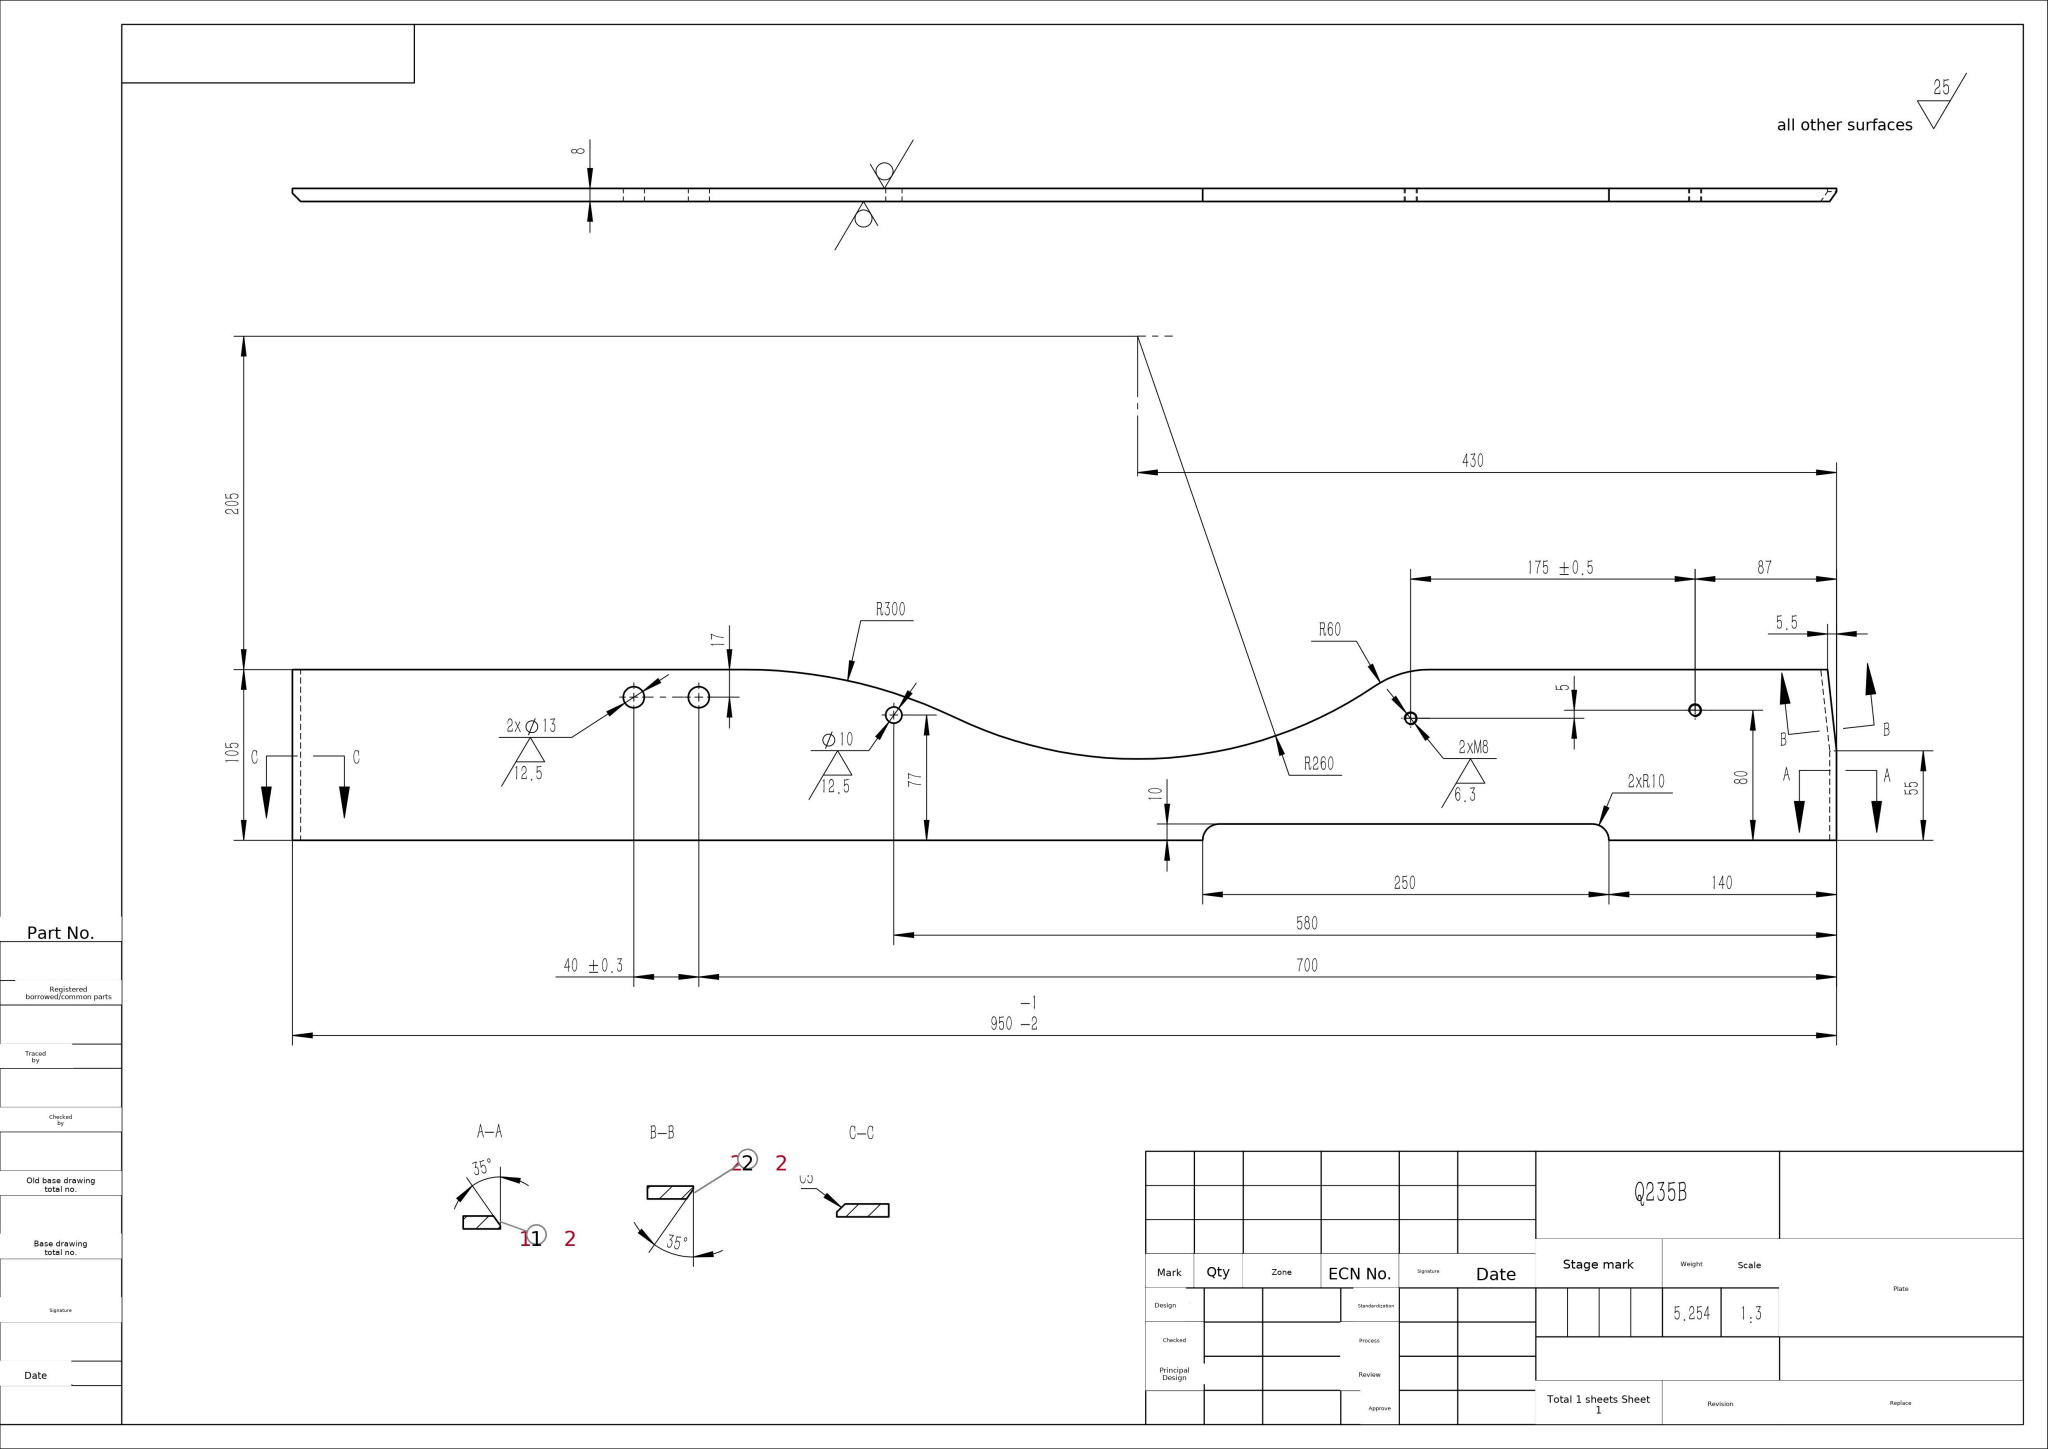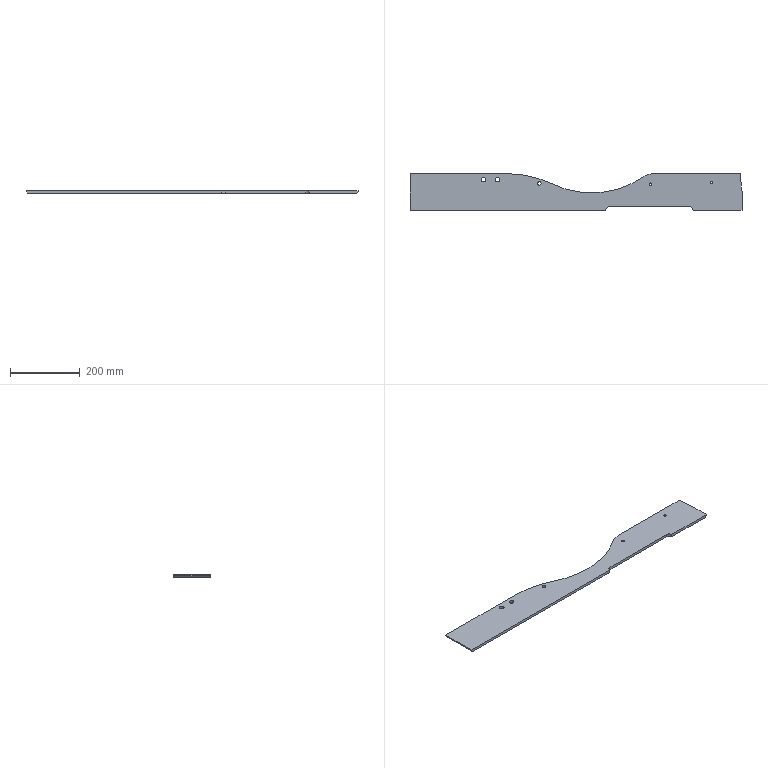Part | SolidWorks | mm | material Q235B | 1 solid | 28 faces | box 950 x 105 x 8 mm | volume 671051 mm3 | cylinder 15 | plane 13 | commonest cylinder face diameters 6.8 x4 13 x4 10 x2 20 x2 120 x1 520 x1 600 x1
build123d program:
from build123d import *
from OCP.BRepFilletAPI import BRepFilletAPI_MakeChamfer

# Parameters (mm, degrees)
SKETCH1_R           = 5
SKETCH1_R_2         = 6.5
BOSS_EXTRUDE1_DEPTH = 8
M8_TAPPED_HOLE1_D   = 6.8
CHAMFER1_SIZE       = 5
CHAMFER2_SIZE       = 6
CHAMFER2_SIZE2      = 4.201


with BuildPart() as part:
    # Sketch1 → Boss-Extrude1 (new body)
    with BuildSketch(Plane.XY):
        with BuildLine():
            Line((0, 0), (560, 0))
            ThreePointArc((560, 0), (562.929, 7.071), (570, 10))
            Line((570, 10), (800, 10))
            ThreePointArc((800, 10), (807.071, 7.071), (810, 0))
            Line((810, 0), (950, 0))
            Line((950, 0), (950, 55))
            Line((950, 55), (944.5, 105))
            Line((944.5, 105), (699.374, 105))
            ThreePointArc((699.374, 105), (681.785, 102.364), (665.741, 94.688))
            ThreePointArc((665.741, 94.688), (539.239, 50.713), (407.632, 75.536))
            ThreePointArc((407.632, 75.536), (344.458, 97.541), (277.977, 105))
            Line((277.977, 105), (0, 105))
            Line((0, 105), (0, 0))
        make_face()
        with Locations((370, 77)):
            Circle(SKETCH1_R, mode=Mode.SUBTRACT)
        with Locations((250, 88)):
            Circle(SKETCH1_R_2, mode=Mode.SUBTRACT)
        with Locations((210, 88)):
            Circle(SKETCH1_R_2, mode=Mode.SUBTRACT)
    extrude(amount=BOSS_EXTRUDE1_DEPTH)

    # M8 Tapped Hole1 (through all)
    with Locations(Plane(origin=(863, 80, 8), x_dir=(1, 0, 0), z_dir=(0, 0, 1))):
        with Locations((0, 0), (-175, -5)):
            Hole(M8_TAPPED_HOLE1_D / 2)

    # Chamfer1
    chamfer1_edges = [part.edges().sort_by_distance(p)[0] for p in [
        (0, 52.5, 0),
    ]]
    chamfer(chamfer1_edges, length=CHAMFER1_SIZE)

    # Chamfer2: one chamfer whose edges measure the first distance from different faces: ONE call of the kernel's chamfer builder (chamfer() names one face for all edges)
    chamfer2_edges_1 = [part.edges().sort_by_distance(p)[0] for p in [
        (947.25, 80, 0),
    ]]
    chamfer2_side_1 = [part.faces().sort_by_distance(p)[0] for p in [
        (947.25, 80, 4),
    ]]
    chamfer2_edges_2 = [part.edges().sort_by_distance(p)[0] for p in [
        (950, 27.5, 0),
    ]]
    chamfer2_side_2 = [part.faces().sort_by_distance(p)[0] for p in [
        (950, 27.5, 4),
    ]]
    chamfer2 = BRepFilletAPI_MakeChamfer(part.part.solid().wrapped)
    for e in chamfer2_edges_1:
        chamfer2.Add(CHAMFER2_SIZE, CHAMFER2_SIZE2, e.wrapped, chamfer2_side_1[0].wrapped)  # the first distance lies on this face
    for e in chamfer2_edges_2:
        chamfer2.Add(CHAMFER2_SIZE, CHAMFER2_SIZE2, e.wrapped, chamfer2_side_2[0].wrapped)  # the first distance lies on this face
    add(Compound.cast(chamfer2.Shape()), mode=Mode.REPLACE)


solid = part.part
STEP:
#1=CARTESIAN_POINT('',(866.4,80.,0.));
#2=VERTEX_POINT('',#1);
#3=CARTESIAN_POINT('',(859.6,80.,0.));
#4=VERTEX_POINT('',#3);
#5=CARTESIAN_POINT('',(863.,80.,0.));
#6=DIRECTION('',(0.,0.,-1.));
#7=DIRECTION('',(-1.,0.,0.));
#8=AXIS2_PLACEMENT_3D('',#5,#6,#7);
#9=CIRCLE('',#8,3.4);
#10=EDGE_CURVE('',#2,#4,#9,.T.);
#11=ORIENTED_EDGE('',*,*,#10,.T.);
#12=CARTESIAN_POINT('',(859.6,80.,8.));
#13=VERTEX_POINT('',#12);
#14=CARTESIAN_POINT('',(859.6,80.,8.));
#15=DIRECTION('',(0.,0.,1.));
#16=VECTOR('',#15,1000.);
#17=LINE('',#14,#16);
#18=EDGE_CURVE('',#4,#13,#17,.T.);
#19=ORIENTED_EDGE('',*,*,#18,.T.);
#20=CARTESIAN_POINT('',(866.4,80.,8.));
#21=VERTEX_POINT('',#20);
#22=CARTESIAN_POINT('',(863.,80.,8.));
#23=DIRECTION('',(0.,0.,1.));
#24=DIRECTION('',(1.,0.,0.));
#25=AXIS2_PLACEMENT_3D('',#22,#23,#24);
#26=CIRCLE('',#25,3.4);
#27=EDGE_CURVE('',#13,#21,#26,.T.);
#28=ORIENTED_EDGE('',*,*,#27,.T.);
#29=CARTESIAN_POINT('',(866.4,80.,8.));
#30=DIRECTION('',(0.,0.,1.));
#31=VECTOR('',#30,1000.);
#32=LINE('',#29,#31);
#33=EDGE_CURVE('',#2,#21,#32,.T.);
#34=ORIENTED_EDGE('',*,*,#33,.F.);
#35=EDGE_LOOP('',(#11,#19,#28,#34));
#36=FACE_OUTER_BOUND('',#35,.T.);
#37=CARTESIAN_POINT('',(863.,80.,8.));
#38=DIRECTION('',(0.,0.,1.));
#39=DIRECTION('',(1.,0.,0.));
#40=AXIS2_PLACEMENT_3D('',#37,#38,#39);
#41=CYLINDRICAL_SURFACE('',#40,3.4);
#42=ADVANCED_FACE('',(#36),#41,.F.);
#43=CARTESIAN_POINT('',(691.4,75.,0.));
#44=VERTEX_POINT('',#43);
#45=CARTESIAN_POINT('',(684.6,75.,0.));
#46=VERTEX_POINT('',#45);
#47=CARTESIAN_POINT('',(688.,75.,0.));
#48=DIRECTION('',(0.,0.,-1.));
#49=DIRECTION('',(-1.,0.,0.));
#50=AXIS2_PLACEMENT_3D('',#47,#48,#49);
#51=CIRCLE('',#50,3.4);
#52=EDGE_CURVE('',#44,#46,#51,.T.);
#53=ORIENTED_EDGE('',*,*,#52,.T.);
#54=CARTESIAN_POINT('',(684.6,75.,8.));
#55=VERTEX_POINT('',#54);
#56=CARTESIAN_POINT('',(684.6,75.,8.));
#57=DIRECTION('',(0.,0.,1.));
#58=VECTOR('',#57,1000.);
#59=LINE('',#56,#58);
#60=EDGE_CURVE('',#46,#55,#59,.T.);
#61=ORIENTED_EDGE('',*,*,#60,.T.);
#62=CARTESIAN_POINT('',(691.4,75.,8.));
#63=VERTEX_POINT('',#62);
#64=CARTESIAN_POINT('',(688.,75.,8.));
#65=DIRECTION('',(0.,0.,1.));
#66=DIRECTION('',(1.,0.,0.));
#67=AXIS2_PLACEMENT_3D('',#64,#65,#66);
#68=CIRCLE('',#67,3.4);
#69=EDGE_CURVE('',#55,#63,#68,.T.);
#70=ORIENTED_EDGE('',*,*,#69,.T.);
#71=CARTESIAN_POINT('',(691.4,75.,8.));
#72=DIRECTION('',(0.,0.,1.));
#73=VECTOR('',#72,1000.);
#74=LINE('',#71,#73);
#75=EDGE_CURVE('',#44,#63,#74,.T.);
#76=ORIENTED_EDGE('',*,*,#75,.F.);
#77=EDGE_LOOP('',(#53,#61,#70,#76));
#78=FACE_OUTER_BOUND('',#77,.T.);
#79=CARTESIAN_POINT('',(688.,75.,8.));
#80=DIRECTION('',(0.,0.,1.));
#81=DIRECTION('',(1.,0.,0.));
#82=AXIS2_PLACEMENT_3D('',#79,#80,#81);
#83=CYLINDRICAL_SURFACE('',#82,3.4);
#84=ADVANCED_FACE('',(#78),#83,.F.);
#85=CARTESIAN_POINT('',(203.5,88.,8.));
#86=VERTEX_POINT('',#85);
#87=CARTESIAN_POINT('',(216.5,88.,8.));
#88=VERTEX_POINT('',#87);
#89=CARTESIAN_POINT('',(210.,88.,8.));
#90=DIRECTION('',(0.,0.,1.));
#91=DIRECTION('',(1.,0.,0.));
#92=AXIS2_PLACEMENT_3D('',#89,#90,#91);
#93=CIRCLE('',#92,6.5);
#94=EDGE_CURVE('',#86,#88,#93,.T.);
#95=ORIENTED_EDGE('',*,*,#94,.T.);
#96=CARTESIAN_POINT('',(216.5,88.,0.));
#97=VERTEX_POINT('',#96);
#98=CARTESIAN_POINT('',(216.5,88.,8.));
#99=DIRECTION('',(0.,0.,-1.));
#100=VECTOR('',#99,1000.);
#101=LINE('',#98,#100);
#102=EDGE_CURVE('',#88,#97,#101,.T.);
#103=ORIENTED_EDGE('',*,*,#102,.T.);
#104=CARTESIAN_POINT('',(203.5,88.,0.));
#105=VERTEX_POINT('',#104);
#106=CARTESIAN_POINT('',(210.,88.,0.));
#107=DIRECTION('',(0.,0.,1.));
#108=DIRECTION('',(1.,0.,0.));
#109=AXIS2_PLACEMENT_3D('',#106,#107,#108);
#110=CIRCLE('',#109,6.5);
#111=EDGE_CURVE('',#105,#97,#110,.T.);
#112=ORIENTED_EDGE('',*,*,#111,.F.);
#113=CARTESIAN_POINT('',(203.5,88.,8.));
#114=DIRECTION('',(0.,0.,-1.));
#115=VECTOR('',#114,1000.);
#116=LINE('',#113,#115);
#117=EDGE_CURVE('',#86,#105,#116,.T.);
#118=ORIENTED_EDGE('',*,*,#117,.F.);
#119=EDGE_LOOP('',(#95,#103,#112,#118));
#120=FACE_OUTER_BOUND('',#119,.T.);
#121=CARTESIAN_POINT('',(210.,88.,8.));
#122=DIRECTION('',(0.,0.,-1.));
#123=DIRECTION('',(-1.,0.,0.));
#124=AXIS2_PLACEMENT_3D('',#121,#122,#123);
#125=CYLINDRICAL_SURFACE('',#124,6.5);
#126=ADVANCED_FACE('',(#120),#125,.F.);
#127=CARTESIAN_POINT('',(243.5,88.,8.));
#128=VERTEX_POINT('',#127);
#129=CARTESIAN_POINT('',(256.5,88.,8.));
#130=VERTEX_POINT('',#129);
#131=CARTESIAN_POINT('',(250.,88.,8.));
#132=DIRECTION('',(0.,0.,1.));
#133=DIRECTION('',(1.,0.,0.));
#134=AXIS2_PLACEMENT_3D('',#131,#132,#133);
#135=CIRCLE('',#134,6.5);
#136=EDGE_CURVE('',#128,#130,#135,.T.);
#137=ORIENTED_EDGE('',*,*,#136,.T.);
#138=CARTESIAN_POINT('',(256.5,88.,0.));
#139=VERTEX_POINT('',#138);
#140=CARTESIAN_POINT('',(256.5,88.,8.));
#141=DIRECTION('',(0.,0.,-1.));
#142=VECTOR('',#141,1000.);
#143=LINE('',#140,#142);
#144=EDGE_CURVE('',#130,#139,#143,.T.);
#145=ORIENTED_EDGE('',*,*,#144,.T.);
#146=CARTESIAN_POINT('',(243.5,88.,0.));
#147=VERTEX_POINT('',#146);
#148=CARTESIAN_POINT('',(250.,88.,0.));
#149=DIRECTION('',(0.,0.,1.));
#150=DIRECTION('',(1.,0.,0.));
#151=AXIS2_PLACEMENT_3D('',#148,#149,#150);
#152=CIRCLE('',#151,6.5);
#153=EDGE_CURVE('',#147,#139,#152,.T.);
#154=ORIENTED_EDGE('',*,*,#153,.F.);
#155=CARTESIAN_POINT('',(243.5,88.,8.));
#156=DIRECTION('',(0.,0.,-1.));
#157=VECTOR('',#156,1000.);
#158=LINE('',#155,#157);
#159=EDGE_CURVE('',#128,#147,#158,.T.);
#160=ORIENTED_EDGE('',*,*,#159,.F.);
#161=EDGE_LOOP('',(#137,#145,#154,#160));
#162=FACE_OUTER_BOUND('',#161,.T.);
#163=CARTESIAN_POINT('',(250.,88.,8.));
#164=DIRECTION('',(0.,0.,-1.));
#165=DIRECTION('',(-1.,0.,0.));
#166=AXIS2_PLACEMENT_3D('',#163,#164,#165);
#167=CYLINDRICAL_SURFACE('',#166,6.5);
#168=ADVANCED_FACE('',(#162),#167,.F.);
#169=CARTESIAN_POINT('',(365.,77.,8.));
#170=VERTEX_POINT('',#169);
#171=CARTESIAN_POINT('',(375.,77.,8.));
#172=VERTEX_POINT('',#171);
#173=CARTESIAN_POINT('',(370.,77.,8.));
#174=DIRECTION('',(0.,0.,1.));
#175=DIRECTION('',(1.,0.,0.));
#176=AXIS2_PLACEMENT_3D('',#173,#174,#175);
#177=CIRCLE('',#176,5.);
#178=EDGE_CURVE('',#170,#172,#177,.T.);
#179=ORIENTED_EDGE('',*,*,#178,.T.);
#180=CARTESIAN_POINT('',(375.,77.,0.));
#181=VERTEX_POINT('',#180);
#182=CARTESIAN_POINT('',(375.,77.,8.));
#183=DIRECTION('',(0.,0.,-1.));
#184=VECTOR('',#183,1000.);
#185=LINE('',#182,#184);
#186=EDGE_CURVE('',#172,#181,#185,.T.);
#187=ORIENTED_EDGE('',*,*,#186,.T.);
#188=CARTESIAN_POINT('',(365.,77.,0.));
#189=VERTEX_POINT('',#188);
#190=CARTESIAN_POINT('',(370.,77.,0.));
#191=DIRECTION('',(0.,0.,1.));
#192=DIRECTION('',(1.,0.,0.));
#193=AXIS2_PLACEMENT_3D('',#190,#191,#192);
#194=CIRCLE('',#193,5.);
#195=EDGE_CURVE('',#189,#181,#194,.T.);
#196=ORIENTED_EDGE('',*,*,#195,.F.);
#197=CARTESIAN_POINT('',(365.,77.,8.));
#198=DIRECTION('',(0.,0.,-1.));
#199=VECTOR('',#198,1000.);
#200=LINE('',#197,#199);
#201=EDGE_CURVE('',#170,#189,#200,.T.);
#202=ORIENTED_EDGE('',*,*,#201,.F.);
#203=EDGE_LOOP('',(#179,#187,#196,#202));
#204=FACE_OUTER_BOUND('',#203,.T.);
#205=CARTESIAN_POINT('',(370.,77.,8.));
#206=DIRECTION('',(0.,0.,-1.));
#207=DIRECTION('',(-1.,0.,0.));
#208=AXIS2_PLACEMENT_3D('',#205,#206,#207);
#209=CYLINDRICAL_SURFACE('',#208,5.);
#210=ADVANCED_FACE('',(#204),#209,.F.);
#211=CARTESIAN_POINT('',(0.,105.,8.));
#212=VERTEX_POINT('',#211);
#213=CARTESIAN_POINT('',(0.,0.,8.));
#214=VERTEX_POINT('',#213);
#215=CARTESIAN_POINT('',(0.,105.,8.));
#216=DIRECTION('',(0.,-1.,0.));
#217=VECTOR('',#216,1000.);
#218=LINE('',#215,#217);
#219=EDGE_CURVE('',#212,#214,#218,.T.);
#220=ORIENTED_EDGE('',*,*,#219,.T.);
#221=CARTESIAN_POINT('',(560.,0.,8.));
#222=VERTEX_POINT('',#221);
#223=CARTESIAN_POINT('',(0.,0.,8.));
#224=DIRECTION('',(1.,0.,0.));
#225=VECTOR('',#224,1000.);
#226=LINE('',#223,#225);
#227=EDGE_CURVE('',#214,#222,#226,.T.);
#228=ORIENTED_EDGE('',*,*,#227,.T.);
#229=CARTESIAN_POINT('',(570.,10.,8.));
#230=VERTEX_POINT('',#229);
#231=CARTESIAN_POINT('',(570.,0.,8.));
#232=DIRECTION('',(0.,0.,-1.));
#233=DIRECTION('',(-1.,0.,0.));
#234=AXIS2_PLACEMENT_3D('',#231,#232,#233);
#235=CIRCLE('',#234,10.);
#236=EDGE_CURVE('',#222,#230,#235,.T.);
#237=ORIENTED_EDGE('',*,*,#236,.T.);
#238=CARTESIAN_POINT('',(800.,10.,8.));
#239=VERTEX_POINT('',#238);
#240=CARTESIAN_POINT('',(570.,10.,8.));
#241=DIRECTION('',(1.,0.,0.));
#242=VECTOR('',#241,1000.);
#243=LINE('',#240,#242);
#244=EDGE_CURVE('',#230,#239,#243,.T.);
#245=ORIENTED_EDGE('',*,*,#244,.T.);
#246=CARTESIAN_POINT('',(810.,0.,8.));
#247=VERTEX_POINT('',#246);
#248=CARTESIAN_POINT('',(800.,-0.,8.));
#249=DIRECTION('',(0.,0.,-1.));
#250=DIRECTION('',(1.,0.,0.));
#251=AXIS2_PLACEMENT_3D('',#248,#249,#250);
#252=CIRCLE('',#251,10.);
#253=EDGE_CURVE('',#239,#247,#252,.T.);
#254=ORIENTED_EDGE('',*,*,#253,.T.);
#255=CARTESIAN_POINT('',(950.,0.,8.));
#256=VERTEX_POINT('',#255);
#257=CARTESIAN_POINT('',(810.,0.,8.));
#258=DIRECTION('',(1.,0.,0.));
#259=VECTOR('',#258,1000.);
#260=LINE('',#257,#259);
#261=EDGE_CURVE('',#247,#256,#260,.T.);
#262=ORIENTED_EDGE('',*,*,#261,.T.);
#263=CARTESIAN_POINT('',(950.,55.,8.));
#264=VERTEX_POINT('',#263);
#265=CARTESIAN_POINT('',(950.,0.,8.));
#266=DIRECTION('',(0.,1.,0.));
#267=VECTOR('',#266,1000.);
#268=LINE('',#265,#267);
#269=EDGE_CURVE('',#256,#264,#268,.T.);
#270=ORIENTED_EDGE('',*,*,#269,.T.);
#271=CARTESIAN_POINT('',(944.5,105.,8.));
#272=VERTEX_POINT('',#271);
#273=CARTESIAN_POINT('',(950.,55.,8.));
#274=DIRECTION('',(-0.1093,0.994,0.));
#275=VECTOR('',#274,1000.);
#276=LINE('',#273,#275);
#277=EDGE_CURVE('',#264,#272,#276,.T.);
#278=ORIENTED_EDGE('',*,*,#277,.T.);
#279=CARTESIAN_POINT('',(699.374,105.,8.));
#280=VERTEX_POINT('',#279);
#281=CARTESIAN_POINT('',(944.5,105.,8.));
#282=DIRECTION('',(-1.,-0.,0.));
#283=VECTOR('',#282,1000.);
#284=LINE('',#281,#283);
#285=EDGE_CURVE('',#272,#280,#284,.T.);
#286=ORIENTED_EDGE('',*,*,#285,.T.);
#287=CARTESIAN_POINT('',(665.741,94.687,8.));
#288=VERTEX_POINT('',#287);
#289=CARTESIAN_POINT('',(699.374,45.,8.));
#290=DIRECTION('',(0.,0.,1.));
#291=DIRECTION('',(-1.,0.,0.));
#292=AXIS2_PLACEMENT_3D('',#289,#290,#291);
#293=CIRCLE('',#292,60.);
#294=EDGE_CURVE('',#280,#288,#293,.T.);
#295=ORIENTED_EDGE('',*,*,#294,.T.);
#296=CARTESIAN_POINT('',(407.632,75.536,8.));
#297=VERTEX_POINT('',#296);
#298=CARTESIAN_POINT('',(520.,310.,8.));
#299=DIRECTION('',(0.,0.,-1.));
#300=DIRECTION('',(1.,0.,0.));
#301=AXIS2_PLACEMENT_3D('',#298,#299,#300);
#302=CIRCLE('',#301,260.);
#303=EDGE_CURVE('',#288,#297,#302,.T.);
#304=ORIENTED_EDGE('',*,*,#303,.T.);
#305=CARTESIAN_POINT('',(277.977,105.,8.));
#306=VERTEX_POINT('',#305);
#307=CARTESIAN_POINT('',(277.977,-195.,8.));
#308=DIRECTION('',(0.,0.,1.));
#309=DIRECTION('',(1.,0.,0.));
#310=AXIS2_PLACEMENT_3D('',#307,#308,#309);
#311=CIRCLE('',#310,300.);
#312=EDGE_CURVE('',#297,#306,#311,.T.);
#313=ORIENTED_EDGE('',*,*,#312,.T.);
#314=CARTESIAN_POINT('',(277.977,105.,8.));
#315=DIRECTION('',(-1.,-0.,0.));
#316=VECTOR('',#315,1000.);
#317=LINE('',#314,#316);
#318=EDGE_CURVE('',#306,#212,#317,.T.);
#319=ORIENTED_EDGE('',*,*,#318,.T.);
#320=EDGE_LOOP('',(#220,#228,#237,#245,#254,#262,#270,#278,#286,#295,#304,#313,#319));
#321=FACE_OUTER_BOUND('',#320,.T.);
#322=ORIENTED_EDGE('',*,*,#178,.F.);
#323=CARTESIAN_POINT('',(370.,77.,8.));
#324=DIRECTION('',(0.,0.,1.));
#325=DIRECTION('',(1.,0.,0.));
#326=AXIS2_PLACEMENT_3D('',#323,#324,#325);
#327=CIRCLE('',#326,5.);
#328=EDGE_CURVE('',#172,#170,#327,.T.);
#329=ORIENTED_EDGE('',*,*,#328,.F.);
#330=EDGE_LOOP('',(#322,#329));
#331=FACE_BOUND('',#330,.T.);
#332=ORIENTED_EDGE('',*,*,#136,.F.);
#333=CARTESIAN_POINT('',(250.,88.,8.));
#334=DIRECTION('',(0.,0.,1.));
#335=DIRECTION('',(1.,0.,0.));
#336=AXIS2_PLACEMENT_3D('',#333,#334,#335);
#337=CIRCLE('',#336,6.5);
#338=EDGE_CURVE('',#130,#128,#337,.T.);
#339=ORIENTED_EDGE('',*,*,#338,.F.);
#340=EDGE_LOOP('',(#332,#339));
#341=FACE_BOUND('',#340,.T.);
#342=ORIENTED_EDGE('',*,*,#94,.F.);
#343=CARTESIAN_POINT('',(210.,88.,8.));
#344=DIRECTION('',(0.,0.,1.));
#345=DIRECTION('',(1.,0.,0.));
#346=AXIS2_PLACEMENT_3D('',#343,#344,#345);
#347=CIRCLE('',#346,6.5);
#348=EDGE_CURVE('',#88,#86,#347,.T.);
#349=ORIENTED_EDGE('',*,*,#348,.F.);
#350=EDGE_LOOP('',(#342,#349));
#351=FACE_BOUND('',#350,.T.);
#352=CARTESIAN_POINT('',(688.,75.,8.));
#353=DIRECTION('',(0.,0.,1.));
#354=DIRECTION('',(1.,0.,0.));
#355=AXIS2_PLACEMENT_3D('',#352,#353,#354);
#356=CIRCLE('',#355,3.4);
#357=EDGE_CURVE('',#63,#55,#356,.T.);
#358=ORIENTED_EDGE('',*,*,#357,.F.);
#359=ORIENTED_EDGE('',*,*,#69,.F.);
#360=EDGE_LOOP('',(#358,#359));
#361=FACE_BOUND('',#360,.T.);
#362=CARTESIAN_POINT('',(863.,80.,8.));
#363=DIRECTION('',(0.,0.,1.));
#364=DIRECTION('',(1.,0.,0.));
#365=AXIS2_PLACEMENT_3D('',#362,#363,#364);
#366=CIRCLE('',#365,3.4);
#367=EDGE_CURVE('',#21,#13,#366,.T.);
#368=ORIENTED_EDGE('',*,*,#367,.F.);
#369=ORIENTED_EDGE('',*,*,#27,.F.);
#370=EDGE_LOOP('',(#368,#369));
#371=FACE_BOUND('',#370,.T.);
#372=CARTESIAN_POINT('',(570.,0.,8.));
#373=DIRECTION('',(0.,0.,-1.));
#374=DIRECTION('',(-1.,0.,0.));
#375=AXIS2_PLACEMENT_3D('',#372,#373,#374);
#376=PLANE('',#375);
#377=ADVANCED_FACE('',(#321,#331,#341,#351,#361,#371),#376,.F.);
#378=ORIENTED_EDGE('',*,*,#10,.F.);
#379=CARTESIAN_POINT('',(863.,80.,0.));
#380=DIRECTION('',(0.,0.,-1.));
#381=DIRECTION('',(-1.,0.,0.));
#382=AXIS2_PLACEMENT_3D('',#379,#380,#381);
#383=CIRCLE('',#382,3.4);
#384=EDGE_CURVE('',#4,#2,#383,.T.);
#385=ORIENTED_EDGE('',*,*,#384,.F.);
#386=EDGE_LOOP('',(#378,#385));
#387=FACE_BOUND('',#386,.T.);
#388=ORIENTED_EDGE('',*,*,#52,.F.);
#389=CARTESIAN_POINT('',(688.,75.,0.));
#390=DIRECTION('',(0.,0.,-1.));
#391=DIRECTION('',(-1.,0.,0.));
#392=AXIS2_PLACEMENT_3D('',#389,#390,#391);
#393=CIRCLE('',#392,3.4);
#394=EDGE_CURVE('',#46,#44,#393,.T.);
#395=ORIENTED_EDGE('',*,*,#394,.F.);
#396=EDGE_LOOP('',(#388,#395));
#397=FACE_BOUND('',#396,.T.);
#398=ORIENTED_EDGE('',*,*,#153,.T.);
#399=CARTESIAN_POINT('',(250.,88.,0.));
#400=DIRECTION('',(0.,0.,1.));
#401=DIRECTION('',(1.,0.,0.));
#402=AXIS2_PLACEMENT_3D('',#399,#400,#401);
#403=CIRCLE('',#402,6.5);
#404=EDGE_CURVE('',#139,#147,#403,.T.);
#405=ORIENTED_EDGE('',*,*,#404,.T.);
#406=EDGE_LOOP('',(#398,#405));
#407=FACE_BOUND('',#406,.T.);
#408=CARTESIAN_POINT('',(940.273,105.,0.));
#409=VERTEX_POINT('',#408);
#410=CARTESIAN_POINT('',(699.374,105.,0.));
#411=VERTEX_POINT('',#410);
#412=CARTESIAN_POINT('',(944.5,105.,0.));
#413=DIRECTION('',(-1.,-0.,0.));
#414=VECTOR('',#413,1000.);
#415=LINE('',#412,#414);
#416=EDGE_CURVE('',#409,#411,#415,.T.);
#417=ORIENTED_EDGE('',*,*,#416,.F.);
#418=CARTESIAN_POINT('',(945.799,54.77,0.));
#419=VERTEX_POINT('',#418);
#420=CARTESIAN_POINT('',(945.824,54.541,0.));
#421=DIRECTION('',(0.1093,-0.994,0.));
#422=VECTOR('',#421,1000.);
#423=LINE('',#420,#422);
#424=EDGE_CURVE('',#409,#419,#423,.T.);
#425=ORIENTED_EDGE('',*,*,#424,.T.);
#426=CARTESIAN_POINT('',(945.799,0.,0.));
#427=VERTEX_POINT('',#426);
#428=CARTESIAN_POINT('',(945.799,0.,0.));
#429=DIRECTION('',(0.,-1.,0.));
#430=VECTOR('',#429,1000.);
#431=LINE('',#428,#430);
#432=EDGE_CURVE('',#419,#427,#431,.T.);
#433=ORIENTED_EDGE('',*,*,#432,.T.);
#434=CARTESIAN_POINT('',(810.,0.,0.));
#435=VERTEX_POINT('',#434);
#436=CARTESIAN_POINT('',(810.,0.,0.));
#437=DIRECTION('',(1.,0.,0.));
#438=VECTOR('',#437,1000.);
#439=LINE('',#436,#438);
#440=EDGE_CURVE('',#435,#427,#439,.T.);
#441=ORIENTED_EDGE('',*,*,#440,.F.);
#442=CARTESIAN_POINT('',(800.,10.,0.));
#443=VERTEX_POINT('',#442);
#444=CARTESIAN_POINT('',(800.,-0.,0.));
#445=DIRECTION('',(0.,0.,-1.));
#446=DIRECTION('',(1.,0.,0.));
#447=AXIS2_PLACEMENT_3D('',#444,#445,#446);
#448=CIRCLE('',#447,10.);
#449=EDGE_CURVE('',#443,#435,#448,.T.);
#450=ORIENTED_EDGE('',*,*,#449,.F.);
#451=CARTESIAN_POINT('',(570.,10.,0.));
#452=VERTEX_POINT('',#451);
#453=CARTESIAN_POINT('',(570.,10.,0.));
#454=DIRECTION('',(1.,0.,0.));
#455=VECTOR('',#454,1000.);
#456=LINE('',#453,#455);
#457=EDGE_CURVE('',#452,#443,#456,.T.);
#458=ORIENTED_EDGE('',*,*,#457,.F.);
#459=CARTESIAN_POINT('',(560.,0.,0.));
#460=VERTEX_POINT('',#459);
#461=CARTESIAN_POINT('',(570.,0.,0.));
#462=DIRECTION('',(0.,0.,-1.));
#463=DIRECTION('',(-1.,0.,0.));
#464=AXIS2_PLACEMENT_3D('',#461,#462,#463);
#465=CIRCLE('',#464,10.);
#466=EDGE_CURVE('',#460,#452,#465,.T.);
#467=ORIENTED_EDGE('',*,*,#466,.F.);
#468=CARTESIAN_POINT('',(5.,0.,0.));
#469=VERTEX_POINT('',#468);
#470=CARTESIAN_POINT('',(0.,0.,0.));
#471=DIRECTION('',(1.,0.,0.));
#472=VECTOR('',#471,1000.);
#473=LINE('',#470,#472);
#474=EDGE_CURVE('',#469,#460,#473,.T.);
#475=ORIENTED_EDGE('',*,*,#474,.F.);
#476=CARTESIAN_POINT('',(5.,105.,0.));
#477=VERTEX_POINT('',#476);
#478=CARTESIAN_POINT('',(5.,105.,0.));
#479=DIRECTION('',(0.,1.,0.));
#480=VECTOR('',#479,1000.);
#481=LINE('',#478,#480);
#482=EDGE_CURVE('',#469,#477,#481,.T.);
#483=ORIENTED_EDGE('',*,*,#482,.T.);
#484=CARTESIAN_POINT('',(277.977,105.,0.));
#485=VERTEX_POINT('',#484);
#486=CARTESIAN_POINT('',(277.977,105.,0.));
#487=DIRECTION('',(-1.,-0.,0.));
#488=VECTOR('',#487,1000.);
#489=LINE('',#486,#488);
#490=EDGE_CURVE('',#485,#477,#489,.T.);
#491=ORIENTED_EDGE('',*,*,#490,.F.);
#492=CARTESIAN_POINT('',(407.632,75.536,0.));
#493=VERTEX_POINT('',#492);
#494=CARTESIAN_POINT('',(277.977,-195.,0.));
#495=DIRECTION('',(0.,0.,1.));
#496=DIRECTION('',(1.,0.,0.));
#497=AXIS2_PLACEMENT_3D('',#494,#495,#496);
#498=CIRCLE('',#497,300.);
#499=EDGE_CURVE('',#493,#485,#498,.T.);
#500=ORIENTED_EDGE('',*,*,#499,.F.);
#501=CARTESIAN_POINT('',(665.741,94.687,0.));
#502=VERTEX_POINT('',#501);
#503=CARTESIAN_POINT('',(520.,310.,0.));
#504=DIRECTION('',(0.,0.,-1.));
#505=DIRECTION('',(1.,0.,0.));
#506=AXIS2_PLACEMENT_3D('',#503,#504,#505);
#507=CIRCLE('',#506,260.);
#508=EDGE_CURVE('',#502,#493,#507,.T.);
#509=ORIENTED_EDGE('',*,*,#508,.F.);
#510=CARTESIAN_POINT('',(699.374,45.,0.));
#511=DIRECTION('',(0.,0.,1.));
#512=DIRECTION('',(-1.,0.,0.));
#513=AXIS2_PLACEMENT_3D('',#510,#511,#512);
#514=CIRCLE('',#513,60.);
#515=EDGE_CURVE('',#411,#502,#514,.T.);
#516=ORIENTED_EDGE('',*,*,#515,.F.);
#517=EDGE_LOOP('',(#417,#425,#433,#441,#450,#458,#467,#475,#483,#491,#500,#509,#516));
#518=FACE_OUTER_BOUND('',#517,.T.);
#519=ORIENTED_EDGE('',*,*,#195,.T.);
#520=CARTESIAN_POINT('',(370.,77.,0.));
#521=DIRECTION('',(0.,0.,1.));
#522=DIRECTION('',(1.,0.,0.));
#523=AXIS2_PLACEMENT_3D('',#520,#521,#522);
#524=CIRCLE('',#523,5.);
#525=EDGE_CURVE('',#181,#189,#524,.T.);
#526=ORIENTED_EDGE('',*,*,#525,.T.);
#527=EDGE_LOOP('',(#519,#526));
#528=FACE_BOUND('',#527,.T.);
#529=ORIENTED_EDGE('',*,*,#111,.T.);
#530=CARTESIAN_POINT('',(210.,88.,0.));
#531=DIRECTION('',(0.,0.,1.));
#532=DIRECTION('',(1.,0.,0.));
#533=AXIS2_PLACEMENT_3D('',#530,#531,#532);
#534=CIRCLE('',#533,6.5);
#535=EDGE_CURVE('',#97,#105,#534,.T.);
#536=ORIENTED_EDGE('',*,*,#535,.T.);
#537=EDGE_LOOP('',(#529,#536));
#538=FACE_BOUND('',#537,.T.);
#539=CARTESIAN_POINT('',(570.,0.,0.));
#540=DIRECTION('',(0.,0.,-1.));
#541=DIRECTION('',(-1.,0.,0.));
#542=AXIS2_PLACEMENT_3D('',#539,#540,#541);
#543=PLANE('',#542);
#544=ADVANCED_FACE('',(#387,#397,#407,#518,#528,#538),#543,.T.);
#545=CARTESIAN_POINT('',(0.,105.,5.));
#546=VERTEX_POINT('',#545);
#547=CARTESIAN_POINT('',(0.,105.,8.));
#548=DIRECTION('',(0.,0.,-1.));
#549=VECTOR('',#548,1000.);
#550=LINE('',#547,#549);
#551=EDGE_CURVE('',#212,#546,#550,.T.);
#552=ORIENTED_EDGE('',*,*,#551,.T.);
#553=CARTESIAN_POINT('',(0.,0.,5.));
#554=VERTEX_POINT('',#553);
#555=CARTESIAN_POINT('',(0.,0.,5.));
#556=DIRECTION('',(0.,-1.,0.));
#557=VECTOR('',#556,1000.);
#558=LINE('',#555,#557);
#559=EDGE_CURVE('',#546,#554,#558,.T.);
#560=ORIENTED_EDGE('',*,*,#559,.T.);
#561=CARTESIAN_POINT('',(0.,0.,8.));
#562=DIRECTION('',(0.,0.,-1.));
#563=VECTOR('',#562,1000.);
#564=LINE('',#561,#563);
#565=EDGE_CURVE('',#214,#554,#564,.T.);
#566=ORIENTED_EDGE('',*,*,#565,.F.);
#567=ORIENTED_EDGE('',*,*,#219,.F.);
#568=EDGE_LOOP('',(#552,#560,#566,#567));
#569=FACE_OUTER_BOUND('',#568,.T.);
#570=CARTESIAN_POINT('',(0.,105.,8.));
#571=DIRECTION('',(1.,0.,0.));
#572=DIRECTION('',(0.,0.,-1.));
#573=AXIS2_PLACEMENT_3D('',#570,#571,#572);
#574=PLANE('',#573);
#575=ADVANCED_FACE('',(#569),#574,.F.);
#576=ORIENTED_EDGE('',*,*,#565,.T.);
#577=CARTESIAN_POINT('',(0.,0.,5.));
#578=DIRECTION('',(0.7071,0.,-0.7071));
#579=VECTOR('',#578,1000.);
#580=LINE('',#577,#579);
#581=EDGE_CURVE('',#554,#469,#580,.T.);
#582=ORIENTED_EDGE('',*,*,#581,.T.);
#583=ORIENTED_EDGE('',*,*,#474,.T.);
#584=CARTESIAN_POINT('',(560.,0.,8.));
#585=DIRECTION('',(0.,0.,-1.));
#586=VECTOR('',#585,1000.);
#587=LINE('',#584,#586);
#588=EDGE_CURVE('',#222,#460,#587,.T.);
#589=ORIENTED_EDGE('',*,*,#588,.F.);
#590=ORIENTED_EDGE('',*,*,#227,.F.);
#591=EDGE_LOOP('',(#576,#582,#583,#589,#590));
#592=FACE_OUTER_BOUND('',#591,.T.);
#593=CARTESIAN_POINT('',(0.,0.,8.));
#594=DIRECTION('',(0.,1.,0.));
#595=DIRECTION('',(0.,0.,1.));
#596=AXIS2_PLACEMENT_3D('',#593,#594,#595);
#597=PLANE('',#596);
#598=ADVANCED_FACE('',(#592),#597,.F.);
#599=ORIENTED_EDGE('',*,*,#466,.T.);
#600=CARTESIAN_POINT('',(570.,10.,8.));
#601=DIRECTION('',(0.,0.,-1.));
#602=VECTOR('',#601,1000.);
#603=LINE('',#600,#602);
#604=EDGE_CURVE('',#230,#452,#603,.T.);
#605=ORIENTED_EDGE('',*,*,#604,.F.);
#606=ORIENTED_EDGE('',*,*,#236,.F.);
#607=ORIENTED_EDGE('',*,*,#588,.T.);
#608=EDGE_LOOP('',(#599,#605,#606,#607));
#609=FACE_OUTER_BOUND('',#608,.T.);
#610=CARTESIAN_POINT('',(570.,0.,8.));
#611=DIRECTION('',(0.,0.,-1.));
#612=DIRECTION('',(-1.,0.,0.));
#613=AXIS2_PLACEMENT_3D('',#610,#611,#612);
#614=CYLINDRICAL_SURFACE('',#613,10.);
#615=ADVANCED_FACE('',(#609),#614,.F.);
#616=ORIENTED_EDGE('',*,*,#457,.T.);
#617=CARTESIAN_POINT('',(800.,10.,8.));
#618=DIRECTION('',(0.,0.,-1.));
#619=VECTOR('',#618,1000.);
#620=LINE('',#617,#619);
#621=EDGE_CURVE('',#239,#443,#620,.T.);
#622=ORIENTED_EDGE('',*,*,#621,.F.);
#623=ORIENTED_EDGE('',*,*,#244,.F.);
#624=ORIENTED_EDGE('',*,*,#604,.T.);
#625=EDGE_LOOP('',(#616,#622,#623,#624));
#626=FACE_OUTER_BOUND('',#625,.T.);
#627=CARTESIAN_POINT('',(570.,10.,8.));
#628=DIRECTION('',(0.,1.,0.));
#629=DIRECTION('',(0.,0.,1.));
#630=AXIS2_PLACEMENT_3D('',#627,#628,#629);
#631=PLANE('',#630);
#632=ADVANCED_FACE('',(#626),#631,.F.);
#633=ORIENTED_EDGE('',*,*,#449,.T.);
#634=CARTESIAN_POINT('',(810.,0.,8.));
#635=DIRECTION('',(0.,0.,-1.));
#636=VECTOR('',#635,1000.);
#637=LINE('',#634,#636);
#638=EDGE_CURVE('',#247,#435,#637,.T.);
#639=ORIENTED_EDGE('',*,*,#638,.F.);
#640=ORIENTED_EDGE('',*,*,#253,.F.);
#641=ORIENTED_EDGE('',*,*,#621,.T.);
#642=EDGE_LOOP('',(#633,#639,#640,#641));
#643=FACE_OUTER_BOUND('',#642,.T.);
#644=CARTESIAN_POINT('',(800.,-0.,8.));
#645=DIRECTION('',(0.,0.,-1.));
#646=DIRECTION('',(-1.,0.,0.));
#647=AXIS2_PLACEMENT_3D('',#644,#645,#646);
#648=CYLINDRICAL_SURFACE('',#647,10.);
#649=ADVANCED_FACE('',(#643),#648,.F.);
#650=ORIENTED_EDGE('',*,*,#440,.T.);
#651=CARTESIAN_POINT('',(950.,0.,6.));
#652=VERTEX_POINT('',#651);
#653=CARTESIAN_POINT('',(950.,0.,6.));
#654=DIRECTION('',(0.5736,0.,0.8192));
#655=VECTOR('',#654,1000.);
#656=LINE('',#653,#655);
#657=EDGE_CURVE('',#427,#652,#656,.T.);
#658=ORIENTED_EDGE('',*,*,#657,.T.);
#659=CARTESIAN_POINT('',(950.,0.,8.));
#660=DIRECTION('',(0.,0.,-1.));
#661=VECTOR('',#660,1000.);
#662=LINE('',#659,#661);
#663=EDGE_CURVE('',#256,#652,#662,.T.);
#664=ORIENTED_EDGE('',*,*,#663,.F.);
#665=ORIENTED_EDGE('',*,*,#261,.F.);
#666=ORIENTED_EDGE('',*,*,#638,.T.);
#667=EDGE_LOOP('',(#650,#658,#664,#665,#666));
#668=FACE_OUTER_BOUND('',#667,.T.);
#669=CARTESIAN_POINT('',(810.,0.,8.));
#670=DIRECTION('',(0.,1.,0.));
#671=DIRECTION('',(0.,0.,1.));
#672=AXIS2_PLACEMENT_3D('',#669,#670,#671);
#673=PLANE('',#672);
#674=ADVANCED_FACE('',(#668),#673,.F.);
#675=ORIENTED_EDGE('',*,*,#663,.T.);
#676=CARTESIAN_POINT('',(950.,55.,6.));
#677=VERTEX_POINT('',#676);
#678=CARTESIAN_POINT('',(950.,55.,6.));
#679=DIRECTION('',(0.,1.,0.));
#680=VECTOR('',#679,1000.);
#681=LINE('',#678,#680);
#682=EDGE_CURVE('',#652,#677,#681,.T.);
#683=ORIENTED_EDGE('',*,*,#682,.T.);
#684=CARTESIAN_POINT('',(950.,55.,8.));
#685=DIRECTION('',(0.,0.,-1.));
#686=VECTOR('',#685,1000.);
#687=LINE('',#684,#686);
#688=EDGE_CURVE('',#264,#677,#687,.T.);
#689=ORIENTED_EDGE('',*,*,#688,.F.);
#690=ORIENTED_EDGE('',*,*,#269,.F.);
#691=EDGE_LOOP('',(#675,#683,#689,#690));
#692=FACE_OUTER_BOUND('',#691,.T.);
#693=CARTESIAN_POINT('',(950.,0.,8.));
#694=DIRECTION('',(-1.,0.,0.));
#695=DIRECTION('',(0.,0.,1.));
#696=AXIS2_PLACEMENT_3D('',#693,#694,#695);
#697=PLANE('',#696);
#698=ADVANCED_FACE('',(#692),#697,.F.);
#699=ORIENTED_EDGE('',*,*,#688,.T.);
#700=CARTESIAN_POINT('',(944.5,105.,6.));
#701=VERTEX_POINT('',#700);
#702=CARTESIAN_POINT('',(944.5,105.,6.));
#703=DIRECTION('',(-0.1093,0.994,0.));
#704=VECTOR('',#703,1000.);
#705=LINE('',#702,#704);
#706=EDGE_CURVE('',#677,#701,#705,.T.);
#707=ORIENTED_EDGE('',*,*,#706,.T.);
#708=CARTESIAN_POINT('',(944.5,105.,8.));
#709=DIRECTION('',(0.,0.,-1.));
#710=VECTOR('',#709,1000.);
#711=LINE('',#708,#710);
#712=EDGE_CURVE('',#272,#701,#711,.T.);
#713=ORIENTED_EDGE('',*,*,#712,.F.);
#714=ORIENTED_EDGE('',*,*,#277,.F.);
#715=EDGE_LOOP('',(#699,#707,#713,#714));
#716=FACE_OUTER_BOUND('',#715,.T.);
#717=CARTESIAN_POINT('',(950.,55.,8.));
#718=DIRECTION('',(-0.994,-0.1093,0.));
#719=DIRECTION('',(0.1093,-0.994,0.));
#720=AXIS2_PLACEMENT_3D('',#717,#718,#719);
#721=PLANE('',#720);
#722=ADVANCED_FACE('',(#716),#721,.F.);
#723=ORIENTED_EDGE('',*,*,#712,.T.);
#724=CARTESIAN_POINT('',(946.324,105.,8.589));
#725=DIRECTION('',(-0.5759,-0.,-0.8175));
#726=VECTOR('',#725,1000.);
#727=LINE('',#724,#726);
#728=EDGE_CURVE('',#701,#409,#727,.T.);
#729=ORIENTED_EDGE('',*,*,#728,.T.);
#730=ORIENTED_EDGE('',*,*,#416,.T.);
#731=CARTESIAN_POINT('',(699.374,105.,8.));
#732=DIRECTION('',(0.,0.,-1.));
#733=VECTOR('',#732,1000.);
#734=LINE('',#731,#733);
#735=EDGE_CURVE('',#280,#411,#734,.T.);
#736=ORIENTED_EDGE('',*,*,#735,.F.);
#737=ORIENTED_EDGE('',*,*,#285,.F.);
#738=EDGE_LOOP('',(#723,#729,#730,#736,#737));
#739=FACE_OUTER_BOUND('',#738,.T.);
#740=CARTESIAN_POINT('',(944.5,105.,8.));
#741=DIRECTION('',(0.,-1.,0.));
#742=DIRECTION('',(1.,0.,0.));
#743=AXIS2_PLACEMENT_3D('',#740,#741,#742);
#744=PLANE('',#743);
#745=ADVANCED_FACE('',(#739),#744,.F.);
#746=ORIENTED_EDGE('',*,*,#515,.T.);
#747=CARTESIAN_POINT('',(665.741,94.687,8.));
#748=DIRECTION('',(0.,0.,-1.));
#749=VECTOR('',#748,1000.);
#750=LINE('',#747,#749);
#751=EDGE_CURVE('',#288,#502,#750,.T.);
#752=ORIENTED_EDGE('',*,*,#751,.F.);
#753=ORIENTED_EDGE('',*,*,#294,.F.);
#754=ORIENTED_EDGE('',*,*,#735,.T.);
#755=EDGE_LOOP('',(#746,#752,#753,#754));
#756=FACE_OUTER_BOUND('',#755,.T.);
#757=CARTESIAN_POINT('',(699.374,45.,8.));
#758=DIRECTION('',(0.,0.,-1.));
#759=DIRECTION('',(-1.,0.,0.));
#760=AXIS2_PLACEMENT_3D('',#757,#758,#759);
#761=CYLINDRICAL_SURFACE('',#760,60.);
#762=ADVANCED_FACE('',(#756),#761,.T.);
#763=ORIENTED_EDGE('',*,*,#508,.T.);
#764=CARTESIAN_POINT('',(407.632,75.536,8.));
#765=DIRECTION('',(0.,0.,-1.));
#766=VECTOR('',#765,1000.);
#767=LINE('',#764,#766);
#768=EDGE_CURVE('',#297,#493,#767,.T.);
#769=ORIENTED_EDGE('',*,*,#768,.F.);
#770=ORIENTED_EDGE('',*,*,#303,.F.);
#771=ORIENTED_EDGE('',*,*,#751,.T.);
#772=EDGE_LOOP('',(#763,#769,#770,#771));
#773=FACE_OUTER_BOUND('',#772,.T.);
#774=CARTESIAN_POINT('',(520.,310.,8.));
#775=DIRECTION('',(0.,0.,-1.));
#776=DIRECTION('',(-1.,0.,0.));
#777=AXIS2_PLACEMENT_3D('',#774,#775,#776);
#778=CYLINDRICAL_SURFACE('',#777,260.);
#779=ADVANCED_FACE('',(#773),#778,.F.);
#780=ORIENTED_EDGE('',*,*,#499,.T.);
#781=CARTESIAN_POINT('',(277.977,105.,8.));
#782=DIRECTION('',(0.,0.,-1.));
#783=VECTOR('',#782,1000.);
#784=LINE('',#781,#783);
#785=EDGE_CURVE('',#306,#485,#784,.T.);
#786=ORIENTED_EDGE('',*,*,#785,.F.);
#787=ORIENTED_EDGE('',*,*,#312,.F.);
#788=ORIENTED_EDGE('',*,*,#768,.T.);
#789=EDGE_LOOP('',(#780,#786,#787,#788));
#790=FACE_OUTER_BOUND('',#789,.T.);
#791=CARTESIAN_POINT('',(277.977,-195.,8.));
#792=DIRECTION('',(0.,0.,-1.));
#793=DIRECTION('',(-1.,0.,0.));
#794=AXIS2_PLACEMENT_3D('',#791,#792,#793);
#795=CYLINDRICAL_SURFACE('',#794,300.);
#796=ADVANCED_FACE('',(#790),#795,.T.);
#797=ORIENTED_EDGE('',*,*,#490,.T.);
#798=CARTESIAN_POINT('',(0.,105.,5.));
#799=DIRECTION('',(-0.7071,-0.,0.7071));
#800=VECTOR('',#799,1000.);
#801=LINE('',#798,#800);
#802=EDGE_CURVE('',#477,#546,#801,.T.);
#803=ORIENTED_EDGE('',*,*,#802,.T.);
#804=ORIENTED_EDGE('',*,*,#551,.F.);
#805=ORIENTED_EDGE('',*,*,#318,.F.);
#806=ORIENTED_EDGE('',*,*,#785,.T.);
#807=EDGE_LOOP('',(#797,#803,#804,#805,#806));
#808=FACE_OUTER_BOUND('',#807,.T.);
#809=CARTESIAN_POINT('',(277.977,105.,8.));
#810=DIRECTION('',(0.,-1.,0.));
#811=DIRECTION('',(1.,0.,0.));
#812=AXIS2_PLACEMENT_3D('',#809,#810,#811);
#813=PLANE('',#812);
#814=ADVANCED_FACE('',(#808),#813,.F.);
#815=ORIENTED_EDGE('',*,*,#186,.F.);
#816=ORIENTED_EDGE('',*,*,#328,.T.);
#817=ORIENTED_EDGE('',*,*,#201,.T.);
#818=ORIENTED_EDGE('',*,*,#525,.F.);
#819=EDGE_LOOP('',(#815,#816,#817,#818));
#820=FACE_OUTER_BOUND('',#819,.T.);
#821=CARTESIAN_POINT('',(370.,77.,8.));
#822=DIRECTION('',(0.,0.,-1.));
#823=DIRECTION('',(-1.,0.,0.));
#824=AXIS2_PLACEMENT_3D('',#821,#822,#823);
#825=CYLINDRICAL_SURFACE('',#824,5.);
#826=ADVANCED_FACE('',(#820),#825,.F.);
#827=ORIENTED_EDGE('',*,*,#144,.F.);
#828=ORIENTED_EDGE('',*,*,#338,.T.);
#829=ORIENTED_EDGE('',*,*,#159,.T.);
#830=ORIENTED_EDGE('',*,*,#404,.F.);
#831=EDGE_LOOP('',(#827,#828,#829,#830));
#832=FACE_OUTER_BOUND('',#831,.T.);
#833=CARTESIAN_POINT('',(250.,88.,8.));
#834=DIRECTION('',(0.,0.,-1.));
#835=DIRECTION('',(-1.,0.,0.));
#836=AXIS2_PLACEMENT_3D('',#833,#834,#835);
#837=CYLINDRICAL_SURFACE('',#836,6.5);
#838=ADVANCED_FACE('',(#832),#837,.F.);
#839=ORIENTED_EDGE('',*,*,#102,.F.);
#840=ORIENTED_EDGE('',*,*,#348,.T.);
#841=ORIENTED_EDGE('',*,*,#117,.T.);
#842=ORIENTED_EDGE('',*,*,#535,.F.);
#843=EDGE_LOOP('',(#839,#840,#841,#842));
#844=FACE_OUTER_BOUND('',#843,.T.);
#845=CARTESIAN_POINT('',(210.,88.,8.));
#846=DIRECTION('',(0.,0.,-1.));
#847=DIRECTION('',(-1.,0.,0.));
#848=AXIS2_PLACEMENT_3D('',#845,#846,#847);
#849=CYLINDRICAL_SURFACE('',#848,6.5);
#850=ADVANCED_FACE('',(#844),#849,.F.);
#851=ORIENTED_EDGE('',*,*,#60,.F.);
#852=ORIENTED_EDGE('',*,*,#394,.T.);
#853=ORIENTED_EDGE('',*,*,#75,.T.);
#854=ORIENTED_EDGE('',*,*,#357,.T.);
#855=EDGE_LOOP('',(#851,#852,#853,#854));
#856=FACE_OUTER_BOUND('',#855,.T.);
#857=CARTESIAN_POINT('',(688.,75.,8.));
#858=DIRECTION('',(0.,0.,1.));
#859=DIRECTION('',(1.,0.,0.));
#860=AXIS2_PLACEMENT_3D('',#857,#858,#859);
#861=CYLINDRICAL_SURFACE('',#860,3.4);
#862=ADVANCED_FACE('',(#856),#861,.F.);
#863=ORIENTED_EDGE('',*,*,#18,.F.);
#864=ORIENTED_EDGE('',*,*,#384,.T.);
#865=ORIENTED_EDGE('',*,*,#33,.T.);
#866=ORIENTED_EDGE('',*,*,#367,.T.);
#867=EDGE_LOOP('',(#863,#864,#865,#866));
#868=FACE_OUTER_BOUND('',#867,.T.);
#869=CARTESIAN_POINT('',(863.,80.,8.));
#870=DIRECTION('',(0.,0.,1.));
#871=DIRECTION('',(1.,0.,0.));
#872=AXIS2_PLACEMENT_3D('',#869,#870,#871);
#873=CYLINDRICAL_SURFACE('',#872,3.4);
#874=ADVANCED_FACE('',(#868),#873,.F.);
#875=ORIENTED_EDGE('',*,*,#802,.F.);
#876=ORIENTED_EDGE('',*,*,#482,.F.);
#877=ORIENTED_EDGE('',*,*,#581,.F.);
#878=ORIENTED_EDGE('',*,*,#559,.F.);
#879=EDGE_LOOP('',(#875,#876,#877,#878));
#880=FACE_OUTER_BOUND('',#879,.T.);
#881=CARTESIAN_POINT('',(0.,105.,5.));
#882=DIRECTION('',(-0.7071,0.,-0.7071));
#883=DIRECTION('',(0.,1.,0.));
#884=AXIS2_PLACEMENT_3D('',#881,#882,#883);
#885=PLANE('',#884);
#886=ADVANCED_FACE('',(#880),#885,.T.);
#887=ORIENTED_EDGE('',*,*,#657,.F.);
#888=ORIENTED_EDGE('',*,*,#432,.F.);
#889=CARTESIAN_POINT('',(949.009,54.946,4.584));
#890=DIRECTION('',(-0.5733,-0.03144,-0.8187));
#891=VECTOR('',#890,1000.);
#892=LINE('',#889,#891);
#893=EDGE_CURVE('',#677,#419,#892,.T.);
#894=ORIENTED_EDGE('',*,*,#893,.F.);
#895=ORIENTED_EDGE('',*,*,#682,.F.);
#896=EDGE_LOOP('',(#887,#888,#894,#895));
#897=FACE_OUTER_BOUND('',#896,.T.);
#898=CARTESIAN_POINT('',(950.,0.,6.));
#899=DIRECTION('',(0.8192,0.,-0.5736));
#900=DIRECTION('',(0.,-1.,0.));
#901=AXIS2_PLACEMENT_3D('',#898,#899,#900);
#902=PLANE('',#901);
#903=ADVANCED_FACE('',(#897),#902,.T.);
#904=ORIENTED_EDGE('',*,*,#893,.T.);
#905=ORIENTED_EDGE('',*,*,#424,.F.);
#906=ORIENTED_EDGE('',*,*,#728,.F.);
#907=ORIENTED_EDGE('',*,*,#706,.F.);
#908=EDGE_LOOP('',(#904,#905,#906,#907));
#909=FACE_OUTER_BOUND('',#908,.T.);
#910=CARTESIAN_POINT('',(950.,55.,6.));
#911=DIRECTION('',(0.8142,0.08957,-0.5736));
#912=DIRECTION('',(0.1093,-0.994,0.));
#913=AXIS2_PLACEMENT_3D('',#910,#911,#912);
#914=PLANE('',#913);
#915=ADVANCED_FACE('',(#909),#914,.T.);
#916=CLOSED_SHELL('',(#42,#84,#126,#168,#210,#377,#544,#575,#598,#615,#632,#649,#674,#698,#722,#745,#762,#779,#796,#814,#826,#838,#850,#862,#874,#886,#903,#915));
#917=MANIFOLD_SOLID_BREP('',#916);
#918=CARTESIAN_POINT('',(0.,0.,0.));
#919=DIRECTION('',(0.,0.,1.));
#920=DIRECTION('',(1.,0.,0.));
#921=AXIS2_PLACEMENT_3D('',#918,#919,#920);
#922=(LENGTH_UNIT()NAMED_UNIT(*)SI_UNIT(.MILLI.,.METRE.));
#923=UNCERTAINTY_MEASURE_WITH_UNIT(LENGTH_MEASURE(0.00001),#922,'','');
#924=(NAMED_UNIT(*)PLANE_ANGLE_UNIT()SI_UNIT($,.RADIAN.));
#925=(NAMED_UNIT(*)SI_UNIT($,.STERADIAN.)SOLID_ANGLE_UNIT());
#926=(GEOMETRIC_REPRESENTATION_CONTEXT(3)GLOBAL_UNCERTAINTY_ASSIGNED_CONTEXT((#923))GLOBAL_UNIT_ASSIGNED_CONTEXT((#922,#924,#925))REPRESENTATION_CONTEXT('',''));
#927=ADVANCED_BREP_SHAPE_REPRESENTATION('',(#917,#921),#926);